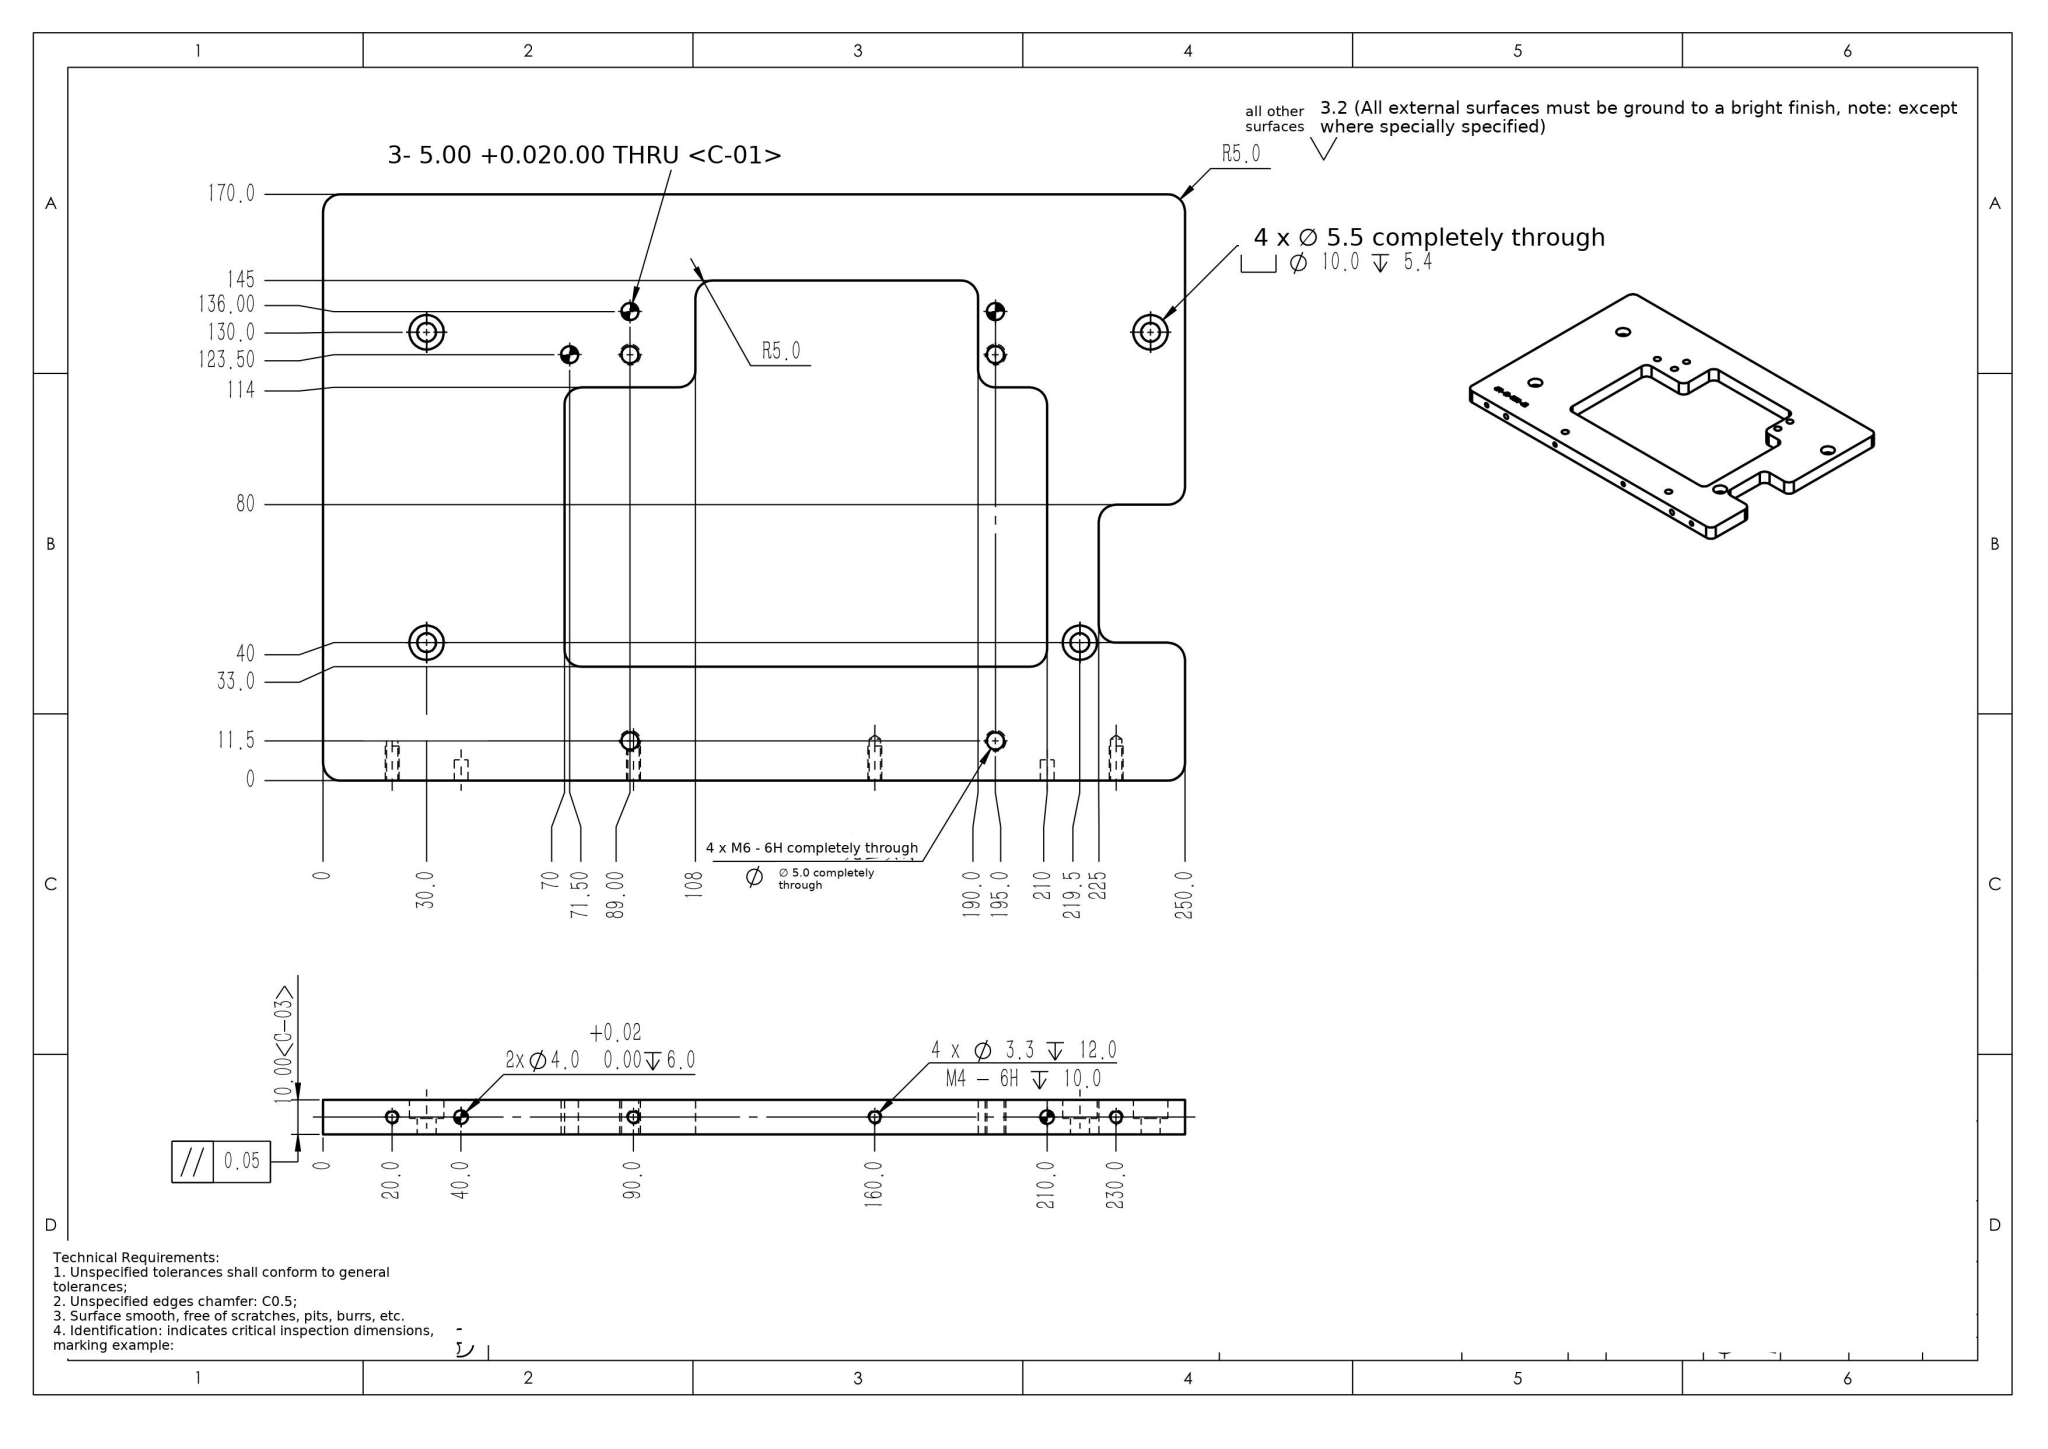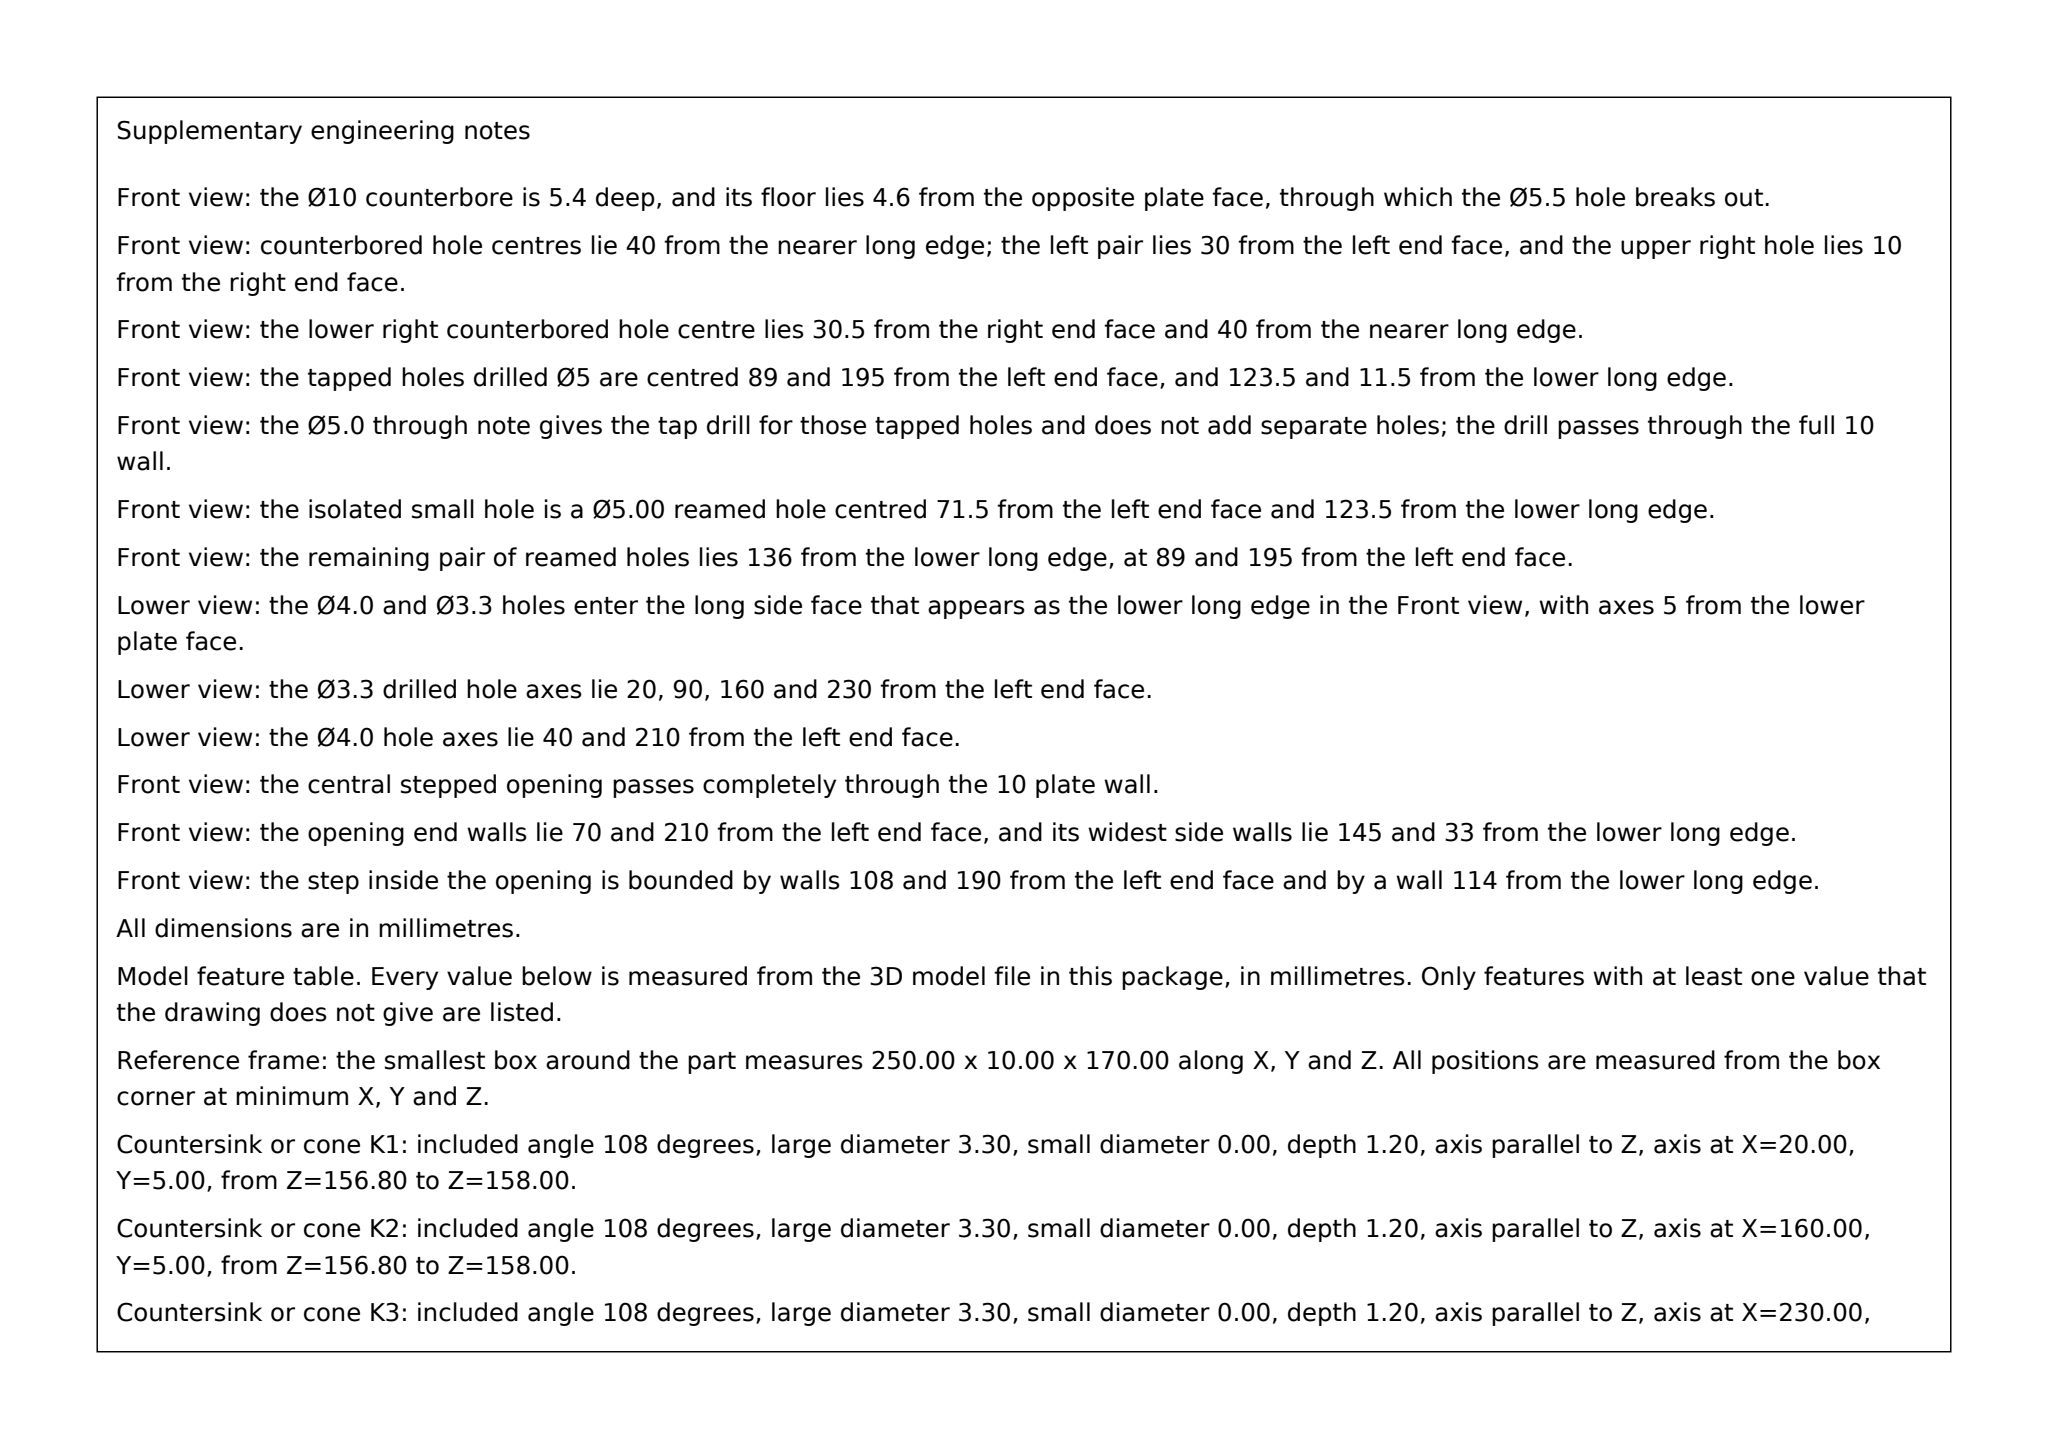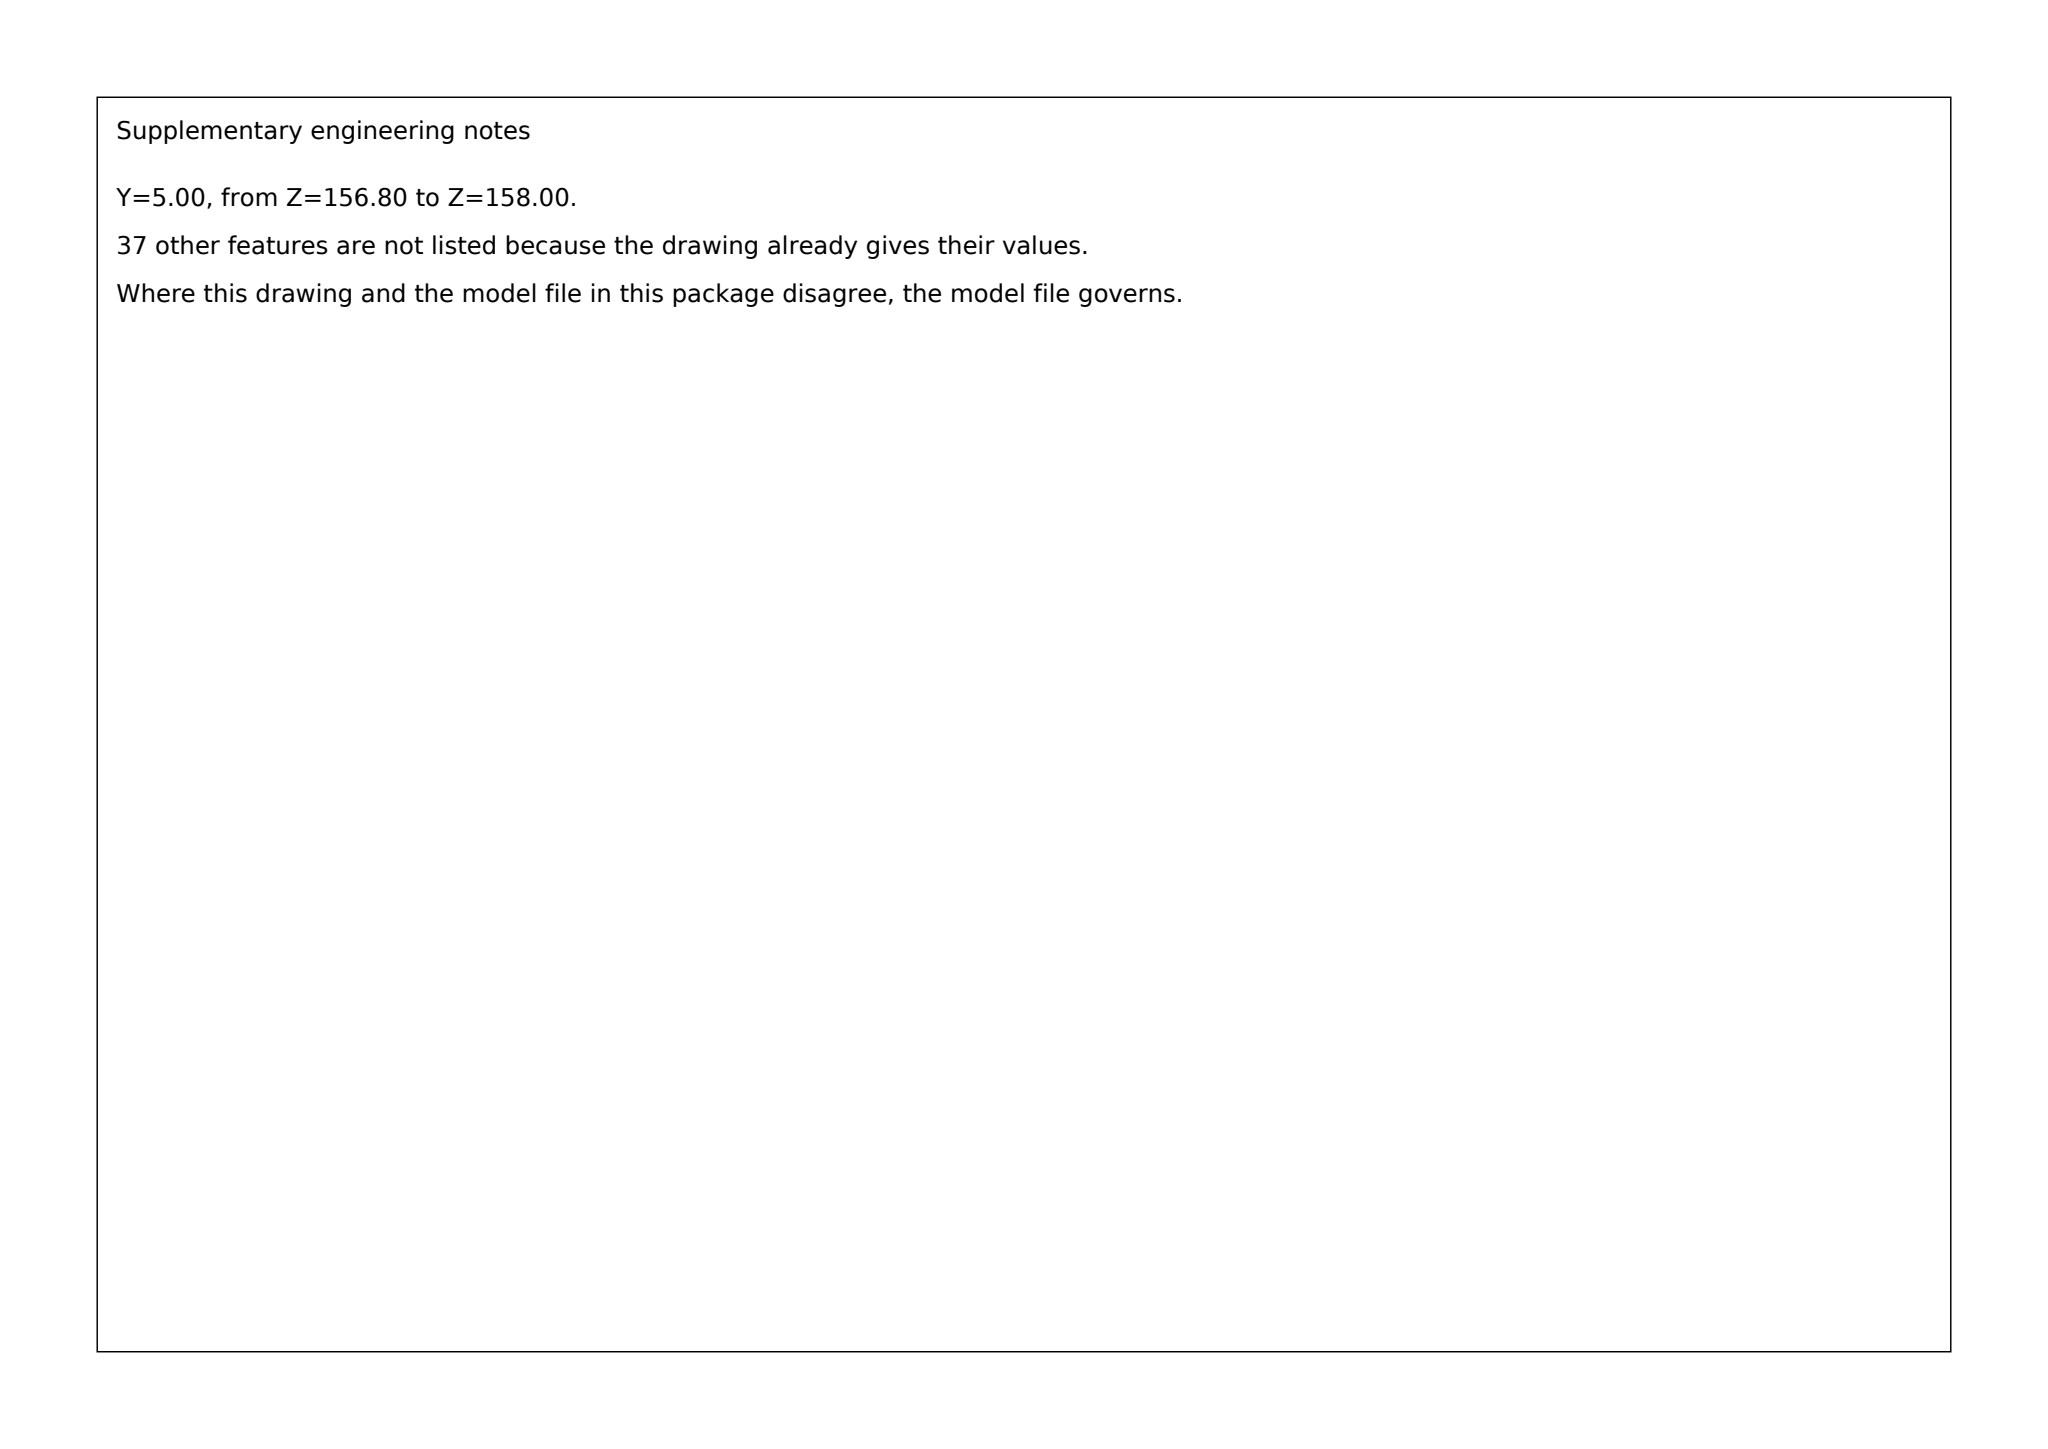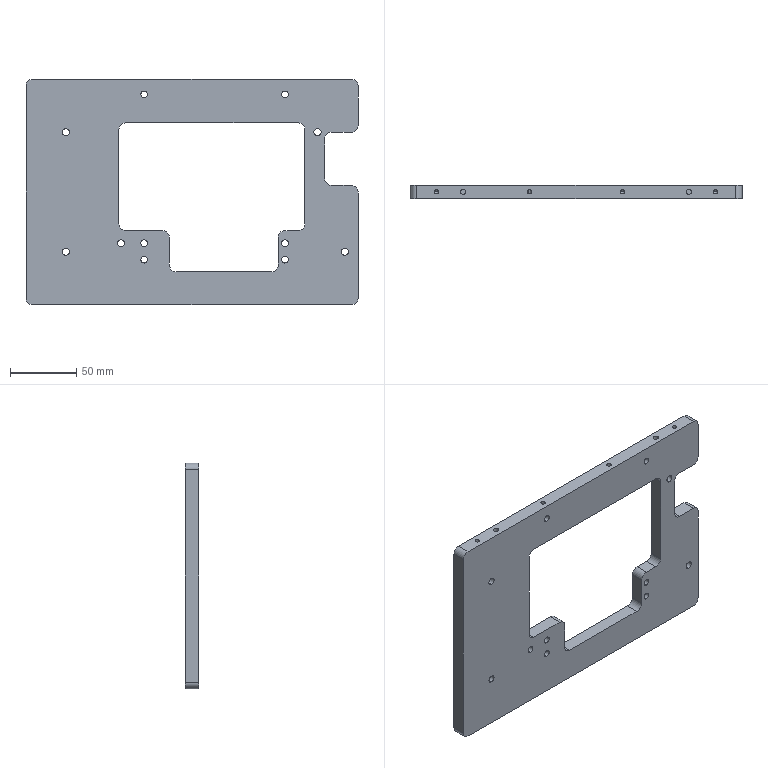Part | SolidWorks | mm | 1 solid | 98 faces | box 250 x 10 x 170 mm | volume 272122 mm3 | cylinder 58 | plane 32 | cone 8 | commonest cylinder face diameters 10 x24 5 x14 5.5 x8 3.3 x8 4 x4
Drawing notes:
PLATE 250 x 170 x 10 THK | from the solid: bbox_xyz 250,10,170; y planes 0 & 10
CENTRAL POCKET 70 TO 210 x 33 TO 114, THRU 10 THK, ALL INT CNRS R5 | from the solid: x planes 70,210; Ø10 y-axis cnr cyls (75,61),(75,132),(205,61),(205,132) len 10 = plate thk; z56/z137 = 114/33 from 170 datum
POCKET STEP 108 TO 190, 114 UP TO 145, CNRS R5, THRU | from the solid: x planes 108,190; Ø10 cnr cyls (103,51),(113,30),(185,30),(195,51) len 10; z25/z56 = 145/114 from 170 datum
RH EDGE NOTCH 225-250 X 40-80: ALL CNRS R5.0 | from the solid: R5 cyls axis y at (230,95),(230,125) int & (245,85),(245,135) ext, planes x=225,250 / z=90,130 (dwg z=170-z)
7 X Ø5.0 THRU AT X71.5,89,195 / Z11.5,123.5,136 - ALL EQUAL SIZE | from the solid: dia5.0 y-axis cyls L=10 at (71.5,46.5),(89,34),(89,46.5),(89,158.5),(195,34),(195,46.5),(195,158.5); dwg z=170-z
OUTER PLATE CORNERS R5.0 TYP 4X | from the solid: Ø10 y-axis cyls, L=10 (full thk) at (5,5),(5,165),(245,5),(245,165) = R5 corners of 250x170 bbox